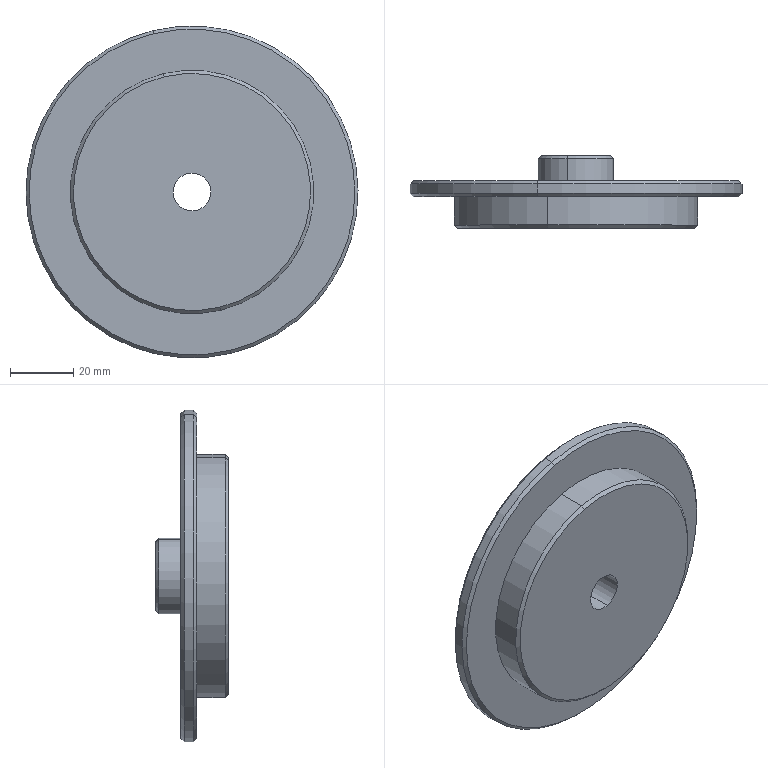Component | SolidWorks | RubberStopWheel-1 | 1 solid | 20 faces | box 105 x 23 x 105 mm | volume 90395 mm3 | cone 8 | cylinder 8 | plane 4 | commonest cylinder face diameters 12 x2 77 x2 105 x2 24 x2
build123d program:
from build123d import *

# Parameters (mm, degrees)
SKETCH1_R           = 12
BOSS_EXTRUDE1_DEPTH = 8
SKETCH2_R           = 52.5
BOSS_EXTRUDE2_DEPTH = 5
SKETCH3_R           = 38.5
BOSS_EXTRUDE3_DEPTH = 10
SKETCH4_R           = 6
CUT_EXTRUDE1_DEPTH  = 99
CHAMFER1_SIZE       = 1


with BuildPart() as part:
    # Sketch1 → Boss-Extrude1 (new body)
    with BuildSketch(Plane.XY):
        Circle(SKETCH1_R)
    extrude(amount=BOSS_EXTRUDE1_DEPTH)

    # Sketch2 → Boss-Extrude2 (add)
    with BuildSketch(Plane.XY.offset(8)):
        Circle(SKETCH2_R)
    extrude(amount=BOSS_EXTRUDE2_DEPTH)

    # Sketch3 → Boss-Extrude3 (add)
    with BuildSketch(Plane.XY.offset(13)):
        Circle(SKETCH3_R)
    extrude(amount=BOSS_EXTRUDE3_DEPTH)

    # Sketch4 → Cut-Extrude1 (cut)
    with BuildSketch(Plane.XY.offset(23)):
        Circle(SKETCH4_R)
    extrude(amount=-CUT_EXTRUDE1_DEPTH, mode=Mode.SUBTRACT)

    # Chamfer1
    chamfer1_edges = [part.edges().sort_by_distance(p)[0] for p in [
        (-38.5, 0, 23),
        (-12, 0, 0),
        (-52.5, 0, 8),
        (-52.5, 0, 13),
    ]]
    chamfer(chamfer1_edges, length=CHAMFER1_SIZE)


solid = part.part

# Placed as in the assembly
solid = solid.moved(Location((-48.547, -49.498, 328), (90, 0, 0)))
STEP:
#1=COLOUR_RGB('',0.7922,0.8196,0.9333);
#2=FILL_AREA_STYLE_COLOUR('',#1);
#3=FILL_AREA_STYLE('',(#2));
#4=SURFACE_STYLE_FILL_AREA(#3);
#5=SURFACE_SIDE_STYLE('',(#4));
#6=SURFACE_STYLE_USAGE(.BOTH.,#5);
#7=PRESENTATION_STYLE_ASSIGNMENT((#6));
#8=CARTESIAN_POINT('',(-1.565,-2.854,11.478));
#9=VERTEX_POINT('',#8);
#10=CARTESIAN_POINT('',(-2.257,-2.854,14.349));
#11=VERTEX_POINT('',#10);
#12=CARTESIAN_POINT('',(-1.911,-2.854,12.913));
#13=DIRECTION('',(0.,-1.,0.));
#14=DIRECTION('',(0.2342,0.,-0.9722));
#15=AXIS2_PLACEMENT_3D('',#12,#13,#14);
#16=CIRCLE('',#15,1.476);
#17=EDGE_CURVE('',#9,#11,#16,.T.);
#18=ORIENTED_EDGE('',*,*,#17,.F.);
#19=CARTESIAN_POINT('',(-1.556,-2.815,11.44));
#20=VERTEX_POINT('',#19);
#21=CARTESIAN_POINT('',(-1.565,-2.854,11.478));
#22=DIRECTION('',(0.1656,0.7071,-0.6874));
#23=VECTOR('',#22,39.37);
#24=LINE('',#21,#23);
#25=EDGE_CURVE('',#9,#20,#24,.T.);
#26=ORIENTED_EDGE('',*,*,#25,.T.);
#27=CARTESIAN_POINT('',(-2.266,-2.815,14.387));
#28=VERTEX_POINT('',#27);
#29=CARTESIAN_POINT('',(-1.911,-2.815,12.913));
#30=DIRECTION('',(-0.,1.,-0.));
#31=DIRECTION('',(0.2342,0.,-0.9722));
#32=AXIS2_PLACEMENT_3D('',#29,#30,#31);
#33=CIRCLE('',#32,1.516);
#34=EDGE_CURVE('',#28,#20,#33,.T.);
#35=ORIENTED_EDGE('',*,*,#34,.F.);
#36=CARTESIAN_POINT('',(-2.257,-2.854,14.349));
#37=DIRECTION('',(-0.1656,0.7071,0.6874));
#38=VECTOR('',#37,39.37);
#39=LINE('',#36,#38);
#40=EDGE_CURVE('',#11,#28,#39,.T.);
#41=ORIENTED_EDGE('',*,*,#40,.F.);
#42=EDGE_LOOP('',(#18,#26,#35,#41));
#43=FACE_OUTER_BOUND('',#42,.T.);
#44=CARTESIAN_POINT('',(-1.911,-2.854,12.913));
#45=DIRECTION('',(-0.,1.,-0.));
#46=DIRECTION('',(-0.2342,0.,0.9722));
#47=AXIS2_PLACEMENT_3D('',#44,#45,#46);
#48=CONICAL_SURFACE('',#47,1.476,0.7854);
#49=ADVANCED_FACE('',(#43),#48,.T.);
#50=CARTESIAN_POINT('',(-2.013,-1.949,13.334));
#51=VERTEX_POINT('',#50);
#52=CARTESIAN_POINT('',(-1.81,-1.949,12.492));
#53=VERTEX_POINT('',#52);
#54=CARTESIAN_POINT('',(-1.911,-1.949,12.913));
#55=DIRECTION('',(-0.,1.,-0.));
#56=DIRECTION('',(0.2342,0.,-0.9722));
#57=AXIS2_PLACEMENT_3D('',#54,#55,#56);
#58=CIRCLE('',#57,0.4331);
#59=EDGE_CURVE('',#51,#53,#58,.T.);
#60=ORIENTED_EDGE('',*,*,#59,.F.);
#61=CARTESIAN_POINT('',(-2.022,-1.988,13.373));
#62=VERTEX_POINT('',#61);
#63=CARTESIAN_POINT('',(-2.022,-1.988,13.373));
#64=DIRECTION('',(-0.1656,-0.7071,0.6874));
#65=VECTOR('',#64,39.37);
#66=LINE('',#63,#65);
#67=EDGE_CURVE('',#51,#62,#66,.T.);
#68=ORIENTED_EDGE('',*,*,#67,.T.);
#69=CARTESIAN_POINT('',(-1.801,-1.988,12.454));
#70=VERTEX_POINT('',#69);
#71=CARTESIAN_POINT('',(-1.911,-1.988,12.913));
#72=DIRECTION('',(0.,-1.,0.));
#73=DIRECTION('',(0.2342,0.,-0.9722));
#74=AXIS2_PLACEMENT_3D('',#71,#72,#73);
#75=CIRCLE('',#74,0.4724);
#76=EDGE_CURVE('',#70,#62,#75,.T.);
#77=ORIENTED_EDGE('',*,*,#76,.F.);
#78=CARTESIAN_POINT('',(-1.801,-1.988,12.454));
#79=DIRECTION('',(0.1656,-0.7071,-0.6874));
#80=VECTOR('',#79,39.37);
#81=LINE('',#78,#80);
#82=EDGE_CURVE('',#53,#70,#81,.T.);
#83=ORIENTED_EDGE('',*,*,#82,.F.);
#84=EDGE_LOOP('',(#60,#68,#77,#83));
#85=FACE_OUTER_BOUND('',#84,.T.);
#86=CARTESIAN_POINT('',(-1.911,-1.988,12.913));
#87=DIRECTION('',(0.,-1.,0.));
#88=DIRECTION('',(0.2342,0.,-0.9722));
#89=AXIS2_PLACEMENT_3D('',#86,#87,#88);
#90=CONICAL_SURFACE('',#89,0.4724,0.7854);
#91=ADVANCED_FACE('',(#85),#90,.T.);
#92=CARTESIAN_POINT('',(-1.436,-2.461,10.942));
#93=VERTEX_POINT('',#92);
#94=CARTESIAN_POINT('',(-2.386,-2.461,14.885));
#95=VERTEX_POINT('',#94);
#96=CARTESIAN_POINT('',(-1.911,-2.461,12.913));
#97=DIRECTION('',(0.,-1.,0.));
#98=DIRECTION('',(0.2342,0.,-0.9722));
#99=AXIS2_PLACEMENT_3D('',#96,#97,#98);
#100=CIRCLE('',#99,2.028);
#101=EDGE_CURVE('',#93,#95,#100,.T.);
#102=ORIENTED_EDGE('',*,*,#101,.F.);
#103=CARTESIAN_POINT('',(-1.427,-2.421,10.904));
#104=VERTEX_POINT('',#103);
#105=CARTESIAN_POINT('',(-1.436,-2.461,10.942));
#106=DIRECTION('',(0.1656,0.7071,-0.6874));
#107=VECTOR('',#106,39.37);
#108=LINE('',#105,#107);
#109=EDGE_CURVE('',#93,#104,#108,.T.);
#110=ORIENTED_EDGE('',*,*,#109,.T.);
#111=CARTESIAN_POINT('',(-2.395,-2.421,14.923));
#112=VERTEX_POINT('',#111);
#113=CARTESIAN_POINT('',(-1.911,-2.421,12.913));
#114=DIRECTION('',(-0.,1.,-0.));
#115=DIRECTION('',(0.2342,0.,-0.9722));
#116=AXIS2_PLACEMENT_3D('',#113,#114,#115);
#117=CIRCLE('',#116,2.067);
#118=EDGE_CURVE('',#112,#104,#117,.T.);
#119=ORIENTED_EDGE('',*,*,#118,.F.);
#120=CARTESIAN_POINT('',(-2.386,-2.461,14.885));
#121=DIRECTION('',(-0.1656,0.7071,0.6874));
#122=VECTOR('',#121,39.37);
#123=LINE('',#120,#122);
#124=EDGE_CURVE('',#95,#112,#123,.T.);
#125=ORIENTED_EDGE('',*,*,#124,.F.);
#126=EDGE_LOOP('',(#102,#110,#119,#125));
#127=FACE_OUTER_BOUND('',#126,.T.);
#128=CARTESIAN_POINT('',(-1.911,-2.461,12.913));
#129=DIRECTION('',(-0.,1.,-0.));
#130=DIRECTION('',(-0.2342,-0.,0.9722));
#131=AXIS2_PLACEMENT_3D('',#128,#129,#130);
#132=CONICAL_SURFACE('',#131,2.028,0.7854);
#133=ADVANCED_FACE('',(#127),#132,.T.);
#134=CARTESIAN_POINT('',(-2.386,-2.264,14.885));
#135=VERTEX_POINT('',#134);
#136=CARTESIAN_POINT('',(-1.436,-2.264,10.942));
#137=VERTEX_POINT('',#136);
#138=CARTESIAN_POINT('',(-1.911,-2.264,12.913));
#139=DIRECTION('',(-0.,1.,-0.));
#140=DIRECTION('',(0.2342,0.,-0.9722));
#141=AXIS2_PLACEMENT_3D('',#138,#139,#140);
#142=CIRCLE('',#141,2.028);
#143=EDGE_CURVE('',#135,#137,#142,.T.);
#144=ORIENTED_EDGE('',*,*,#143,.F.);
#145=CARTESIAN_POINT('',(-2.395,-2.303,14.923));
#146=VERTEX_POINT('',#145);
#147=CARTESIAN_POINT('',(-2.395,-2.303,14.923));
#148=DIRECTION('',(-0.1656,-0.7071,0.6874));
#149=VECTOR('',#148,39.37);
#150=LINE('',#147,#149);
#151=EDGE_CURVE('',#135,#146,#150,.T.);
#152=ORIENTED_EDGE('',*,*,#151,.T.);
#153=CARTESIAN_POINT('',(-1.427,-2.303,10.904));
#154=VERTEX_POINT('',#153);
#155=CARTESIAN_POINT('',(-1.911,-2.303,12.913));
#156=DIRECTION('',(0.,-1.,0.));
#157=DIRECTION('',(0.2342,0.,-0.9722));
#158=AXIS2_PLACEMENT_3D('',#155,#156,#157);
#159=CIRCLE('',#158,2.067);
#160=EDGE_CURVE('',#154,#146,#159,.T.);
#161=ORIENTED_EDGE('',*,*,#160,.F.);
#162=CARTESIAN_POINT('',(-1.427,-2.303,10.904));
#163=DIRECTION('',(0.1656,-0.7071,-0.6874));
#164=VECTOR('',#163,39.37);
#165=LINE('',#162,#164);
#166=EDGE_CURVE('',#137,#154,#165,.T.);
#167=ORIENTED_EDGE('',*,*,#166,.F.);
#168=EDGE_LOOP('',(#144,#152,#161,#167));
#169=FACE_OUTER_BOUND('',#168,.T.);
#170=CARTESIAN_POINT('',(-1.911,-2.303,12.913));
#171=DIRECTION('',(0.,-1.,0.));
#172=DIRECTION('',(0.2342,0.,-0.9722));
#173=AXIS2_PLACEMENT_3D('',#170,#171,#172);
#174=CONICAL_SURFACE('',#173,2.067,0.7854);
#175=ADVANCED_FACE('',(#169),#174,.T.);
#176=CARTESIAN_POINT('',(-1.967,-1.949,13.143));
#177=VERTEX_POINT('',#176);
#178=CARTESIAN_POINT('',(-1.856,-1.949,12.684));
#179=VERTEX_POINT('',#178);
#180=CARTESIAN_POINT('',(-1.911,-1.949,12.913));
#181=DIRECTION('',(0.,-1.,0.));
#182=DIRECTION('',(0.2342,0.,-0.9722));
#183=AXIS2_PLACEMENT_3D('',#180,#181,#182);
#184=CIRCLE('',#183,0.2362);
#185=EDGE_CURVE('',#177,#179,#184,.T.);
#186=ORIENTED_EDGE('',*,*,#185,.F.);
#187=CARTESIAN_POINT('',(-1.967,-2.854,13.143));
#188=VERTEX_POINT('',#187);
#189=CARTESIAN_POINT('',(-1.967,1.043,13.143));
#190=DIRECTION('',(0.,-1.,0.));
#191=VECTOR('',#190,39.37);
#192=LINE('',#189,#191);
#193=EDGE_CURVE('',#177,#188,#192,.T.);
#194=ORIENTED_EDGE('',*,*,#193,.T.);
#195=CARTESIAN_POINT('',(-1.856,-2.854,12.684));
#196=VERTEX_POINT('',#195);
#197=CARTESIAN_POINT('',(-1.911,-2.854,12.913));
#198=DIRECTION('',(0.,-1.,0.));
#199=DIRECTION('',(0.2342,0.,-0.9722));
#200=AXIS2_PLACEMENT_3D('',#197,#198,#199);
#201=CIRCLE('',#200,0.2362);
#202=EDGE_CURVE('',#188,#196,#201,.T.);
#203=ORIENTED_EDGE('',*,*,#202,.T.);
#204=CARTESIAN_POINT('',(-1.856,1.043,12.684));
#205=DIRECTION('',(0.,-1.,0.));
#206=VECTOR('',#205,39.37);
#207=LINE('',#204,#206);
#208=EDGE_CURVE('',#179,#196,#207,.T.);
#209=ORIENTED_EDGE('',*,*,#208,.F.);
#210=EDGE_LOOP('',(#186,#194,#203,#209));
#211=FACE_OUTER_BOUND('',#210,.T.);
#212=CARTESIAN_POINT('',(-1.911,1.043,12.913));
#213=DIRECTION('',(0.,-1.,0.));
#214=DIRECTION('',(0.2342,0.,-0.9722));
#215=AXIS2_PLACEMENT_3D('',#212,#213,#214);
#216=CYLINDRICAL_SURFACE('',#215,0.2362);
#217=ADVANCED_FACE('',(#211),#216,.F.);
#218=ORIENTED_EDGE('',*,*,#34,.T.);
#219=CARTESIAN_POINT('',(-1.556,-2.461,11.44));
#220=VERTEX_POINT('',#219);
#221=CARTESIAN_POINT('',(-1.556,-2.854,11.44));
#222=DIRECTION('',(-0.,1.,-0.));
#223=VECTOR('',#222,39.37);
#224=LINE('',#221,#223);
#225=EDGE_CURVE('',#20,#220,#224,.T.);
#226=ORIENTED_EDGE('',*,*,#225,.T.);
#227=CARTESIAN_POINT('',(-2.266,-2.461,14.387));
#228=VERTEX_POINT('',#227);
#229=CARTESIAN_POINT('',(-1.911,-2.461,12.913));
#230=DIRECTION('',(0.,-1.,0.));
#231=DIRECTION('',(0.2342,0.,-0.9722));
#232=AXIS2_PLACEMENT_3D('',#229,#230,#231);
#233=CIRCLE('',#232,1.516);
#234=EDGE_CURVE('',#220,#228,#233,.T.);
#235=ORIENTED_EDGE('',*,*,#234,.T.);
#236=CARTESIAN_POINT('',(-2.266,-2.854,14.387));
#237=DIRECTION('',(-0.,1.,-0.));
#238=VECTOR('',#237,39.37);
#239=LINE('',#236,#238);
#240=EDGE_CURVE('',#28,#228,#239,.T.);
#241=ORIENTED_EDGE('',*,*,#240,.F.);
#242=EDGE_LOOP('',(#218,#226,#235,#241));
#243=FACE_OUTER_BOUND('',#242,.T.);
#244=CARTESIAN_POINT('',(-1.911,-2.854,12.913));
#245=DIRECTION('',(-0.,1.,-0.));
#246=DIRECTION('',(-0.2342,0.,0.9722));
#247=AXIS2_PLACEMENT_3D('',#244,#245,#246);
#248=CYLINDRICAL_SURFACE('',#247,1.516);
#249=ADVANCED_FACE('',(#243),#248,.T.);
#250=ORIENTED_EDGE('',*,*,#118,.T.);
#251=CARTESIAN_POINT('',(-1.427,-2.461,10.904));
#252=DIRECTION('',(-0.,1.,-0.));
#253=VECTOR('',#252,39.37);
#254=LINE('',#251,#253);
#255=EDGE_CURVE('',#104,#154,#254,.T.);
#256=ORIENTED_EDGE('',*,*,#255,.T.);
#257=ORIENTED_EDGE('',*,*,#160,.T.);
#258=CARTESIAN_POINT('',(-2.395,-2.461,14.923));
#259=DIRECTION('',(-0.,1.,-0.));
#260=VECTOR('',#259,39.37);
#261=LINE('',#258,#260);
#262=EDGE_CURVE('',#112,#146,#261,.T.);
#263=ORIENTED_EDGE('',*,*,#262,.F.);
#264=EDGE_LOOP('',(#250,#256,#257,#263));
#265=FACE_OUTER_BOUND('',#264,.T.);
#266=CARTESIAN_POINT('',(-1.911,-2.461,12.913));
#267=DIRECTION('',(-0.,1.,-0.));
#268=DIRECTION('',(-0.2342,-0.,0.9722));
#269=AXIS2_PLACEMENT_3D('',#266,#267,#268);
#270=CYLINDRICAL_SURFACE('',#269,2.067);
#271=ADVANCED_FACE('',(#265),#270,.T.);
#272=CARTESIAN_POINT('',(-1.801,-2.264,12.454));
#273=VERTEX_POINT('',#272);
#274=CARTESIAN_POINT('',(-2.022,-2.264,13.373));
#275=VERTEX_POINT('',#274);
#276=CARTESIAN_POINT('',(-1.911,-2.264,12.913));
#277=DIRECTION('',(0.,-1.,0.));
#278=DIRECTION('',(0.2342,0.,-0.9722));
#279=AXIS2_PLACEMENT_3D('',#276,#277,#278);
#280=CIRCLE('',#279,0.4724);
#281=EDGE_CURVE('',#273,#275,#280,.T.);
#282=ORIENTED_EDGE('',*,*,#281,.F.);
#283=CARTESIAN_POINT('',(-1.801,-2.264,12.454));
#284=DIRECTION('',(-0.,1.,-0.));
#285=VECTOR('',#284,39.37);
#286=LINE('',#283,#285);
#287=EDGE_CURVE('',#273,#70,#286,.T.);
#288=ORIENTED_EDGE('',*,*,#287,.T.);
#289=ORIENTED_EDGE('',*,*,#76,.T.);
#290=CARTESIAN_POINT('',(-2.022,-2.264,13.373));
#291=DIRECTION('',(-0.,1.,-0.));
#292=VECTOR('',#291,39.37);
#293=LINE('',#290,#292);
#294=EDGE_CURVE('',#275,#62,#293,.T.);
#295=ORIENTED_EDGE('',*,*,#294,.F.);
#296=EDGE_LOOP('',(#282,#288,#289,#295));
#297=FACE_OUTER_BOUND('',#296,.T.);
#298=CARTESIAN_POINT('',(-1.911,-2.264,12.913));
#299=DIRECTION('',(-0.,1.,-0.));
#300=DIRECTION('',(-0.2342,0.,0.9722));
#301=AXIS2_PLACEMENT_3D('',#298,#299,#300);
#302=CYLINDRICAL_SURFACE('',#301,0.4724);
#303=ADVANCED_FACE('',(#297),#302,.T.);
#304=ORIENTED_EDGE('',*,*,#287,.F.);
#305=CARTESIAN_POINT('',(-1.911,-2.264,12.913));
#306=DIRECTION('',(0.,-1.,0.));
#307=DIRECTION('',(0.2342,0.,-0.9722));
#308=AXIS2_PLACEMENT_3D('',#305,#306,#307);
#309=CIRCLE('',#308,0.4724);
#310=EDGE_CURVE('',#275,#273,#309,.T.);
#311=ORIENTED_EDGE('',*,*,#310,.F.);
#312=ORIENTED_EDGE('',*,*,#294,.T.);
#313=CARTESIAN_POINT('',(-1.911,-1.988,12.913));
#314=DIRECTION('',(0.,-1.,0.));
#315=DIRECTION('',(0.2342,0.,-0.9722));
#316=AXIS2_PLACEMENT_3D('',#313,#314,#315);
#317=CIRCLE('',#316,0.4724);
#318=EDGE_CURVE('',#62,#70,#317,.T.);
#319=ORIENTED_EDGE('',*,*,#318,.T.);
#320=EDGE_LOOP('',(#304,#311,#312,#319));
#321=FACE_OUTER_BOUND('',#320,.T.);
#322=CARTESIAN_POINT('',(-1.911,-2.264,12.913));
#323=DIRECTION('',(-0.,1.,-0.));
#324=DIRECTION('',(-0.2342,0.,0.9722));
#325=AXIS2_PLACEMENT_3D('',#322,#323,#324);
#326=CYLINDRICAL_SURFACE('',#325,0.4724);
#327=ADVANCED_FACE('',(#321),#326,.T.);
#328=CARTESIAN_POINT('',(-1.911,-1.949,12.913));
#329=DIRECTION('',(-0.,1.,-0.));
#330=DIRECTION('',(0.2342,0.,-0.9722));
#331=AXIS2_PLACEMENT_3D('',#328,#329,#330);
#332=CIRCLE('',#331,0.4331);
#333=EDGE_CURVE('',#53,#51,#332,.T.);
#334=ORIENTED_EDGE('',*,*,#333,.T.);
#335=ORIENTED_EDGE('',*,*,#59,.T.);
#336=EDGE_LOOP('',(#334,#335));
#337=FACE_OUTER_BOUND('',#336,.T.);
#338=CARTESIAN_POINT('',(-1.911,-1.949,12.913));
#339=DIRECTION('',(0.,-1.,0.));
#340=DIRECTION('',(0.2342,0.,-0.9722));
#341=AXIS2_PLACEMENT_3D('',#338,#339,#340);
#342=CIRCLE('',#341,0.2362);
#343=EDGE_CURVE('',#179,#177,#342,.T.);
#344=ORIENTED_EDGE('',*,*,#343,.T.);
#345=ORIENTED_EDGE('',*,*,#185,.T.);
#346=EDGE_LOOP('',(#344,#345));
#347=FACE_BOUND('',#346,.T.);
#348=CARTESIAN_POINT('',(-1.911,-1.949,12.913));
#349=DIRECTION('',(0.,-1.,0.));
#350=DIRECTION('',(0.2342,0.,-0.9722));
#351=AXIS2_PLACEMENT_3D('',#348,#349,#350);
#352=PLANE('',#351);
#353=ADVANCED_FACE('',(#337,#347),#352,.F.);
#354=ORIENTED_EDGE('',*,*,#255,.F.);
#355=CARTESIAN_POINT('',(-1.911,-2.421,12.913));
#356=DIRECTION('',(-0.,1.,-0.));
#357=DIRECTION('',(0.2342,0.,-0.9722));
#358=AXIS2_PLACEMENT_3D('',#355,#356,#357);
#359=CIRCLE('',#358,2.067);
#360=EDGE_CURVE('',#104,#112,#359,.T.);
#361=ORIENTED_EDGE('',*,*,#360,.T.);
#362=ORIENTED_EDGE('',*,*,#262,.T.);
#363=CARTESIAN_POINT('',(-1.911,-2.303,12.913));
#364=DIRECTION('',(0.,-1.,0.));
#365=DIRECTION('',(0.2342,0.,-0.9722));
#366=AXIS2_PLACEMENT_3D('',#363,#364,#365);
#367=CIRCLE('',#366,2.067);
#368=EDGE_CURVE('',#146,#154,#367,.T.);
#369=ORIENTED_EDGE('',*,*,#368,.T.);
#370=EDGE_LOOP('',(#354,#361,#362,#369));
#371=FACE_OUTER_BOUND('',#370,.T.);
#372=CARTESIAN_POINT('',(-1.911,-2.461,12.913));
#373=DIRECTION('',(-0.,1.,-0.));
#374=DIRECTION('',(-0.2342,-0.,0.9722));
#375=AXIS2_PLACEMENT_3D('',#372,#373,#374);
#376=CYLINDRICAL_SURFACE('',#375,2.067);
#377=ADVANCED_FACE('',(#371),#376,.T.);
#378=CARTESIAN_POINT('',(-1.911,-2.461,12.913));
#379=DIRECTION('',(0.,-1.,0.));
#380=DIRECTION('',(0.2342,0.,-0.9722));
#381=AXIS2_PLACEMENT_3D('',#378,#379,#380);
#382=CIRCLE('',#381,2.028);
#383=EDGE_CURVE('',#95,#93,#382,.T.);
#384=ORIENTED_EDGE('',*,*,#383,.T.);
#385=ORIENTED_EDGE('',*,*,#101,.T.);
#386=EDGE_LOOP('',(#384,#385));
#387=FACE_OUTER_BOUND('',#386,.T.);
#388=CARTESIAN_POINT('',(-1.911,-2.461,12.913));
#389=DIRECTION('',(0.,-1.,0.));
#390=DIRECTION('',(0.2342,0.,-0.9722));
#391=AXIS2_PLACEMENT_3D('',#388,#389,#390);
#392=CIRCLE('',#391,1.516);
#393=EDGE_CURVE('',#228,#220,#392,.T.);
#394=ORIENTED_EDGE('',*,*,#393,.F.);
#395=ORIENTED_EDGE('',*,*,#234,.F.);
#396=EDGE_LOOP('',(#394,#395));
#397=FACE_BOUND('',#396,.T.);
#398=CARTESIAN_POINT('',(-1.911,-2.461,12.913));
#399=DIRECTION('',(0.,-1.,0.));
#400=DIRECTION('',(0.2342,0.,-0.9722));
#401=AXIS2_PLACEMENT_3D('',#398,#399,#400);
#402=PLANE('',#401);
#403=ADVANCED_FACE('',(#387,#397),#402,.T.);
#404=CARTESIAN_POINT('',(-1.911,-2.264,12.913));
#405=DIRECTION('',(-0.,1.,-0.));
#406=DIRECTION('',(0.2342,0.,-0.9722));
#407=AXIS2_PLACEMENT_3D('',#404,#405,#406);
#408=CIRCLE('',#407,2.028);
#409=EDGE_CURVE('',#137,#135,#408,.T.);
#410=ORIENTED_EDGE('',*,*,#409,.T.);
#411=ORIENTED_EDGE('',*,*,#143,.T.);
#412=EDGE_LOOP('',(#410,#411));
#413=FACE_OUTER_BOUND('',#412,.T.);
#414=ORIENTED_EDGE('',*,*,#310,.T.);
#415=ORIENTED_EDGE('',*,*,#281,.T.);
#416=EDGE_LOOP('',(#414,#415));
#417=FACE_BOUND('',#416,.T.);
#418=CARTESIAN_POINT('',(-1.911,-2.264,12.913));
#419=DIRECTION('',(0.,-1.,0.));
#420=DIRECTION('',(0.2342,0.,-0.9722));
#421=AXIS2_PLACEMENT_3D('',#418,#419,#420);
#422=PLANE('',#421);
#423=ADVANCED_FACE('',(#413,#417),#422,.F.);
#424=ORIENTED_EDGE('',*,*,#225,.F.);
#425=CARTESIAN_POINT('',(-1.911,-2.815,12.913));
#426=DIRECTION('',(-0.,1.,-0.));
#427=DIRECTION('',(0.2342,0.,-0.9722));
#428=AXIS2_PLACEMENT_3D('',#425,#426,#427);
#429=CIRCLE('',#428,1.516);
#430=EDGE_CURVE('',#20,#28,#429,.T.);
#431=ORIENTED_EDGE('',*,*,#430,.T.);
#432=ORIENTED_EDGE('',*,*,#240,.T.);
#433=ORIENTED_EDGE('',*,*,#393,.T.);
#434=EDGE_LOOP('',(#424,#431,#432,#433));
#435=FACE_OUTER_BOUND('',#434,.T.);
#436=CARTESIAN_POINT('',(-1.911,-2.854,12.913));
#437=DIRECTION('',(-0.,1.,-0.));
#438=DIRECTION('',(-0.2342,0.,0.9722));
#439=AXIS2_PLACEMENT_3D('',#436,#437,#438);
#440=CYLINDRICAL_SURFACE('',#439,1.516);
#441=ADVANCED_FACE('',(#435),#440,.T.);
#442=CARTESIAN_POINT('',(-1.911,-2.854,12.913));
#443=DIRECTION('',(0.,-1.,0.));
#444=DIRECTION('',(0.2342,0.,-0.9722));
#445=AXIS2_PLACEMENT_3D('',#442,#443,#444);
#446=CIRCLE('',#445,1.476);
#447=EDGE_CURVE('',#11,#9,#446,.T.);
#448=ORIENTED_EDGE('',*,*,#447,.T.);
#449=ORIENTED_EDGE('',*,*,#17,.T.);
#450=EDGE_LOOP('',(#448,#449));
#451=FACE_OUTER_BOUND('',#450,.T.);
#452=CARTESIAN_POINT('',(-1.911,-2.854,12.913));
#453=DIRECTION('',(0.,-1.,0.));
#454=DIRECTION('',(0.2342,0.,-0.9722));
#455=AXIS2_PLACEMENT_3D('',#452,#453,#454);
#456=CIRCLE('',#455,0.2362);
#457=EDGE_CURVE('',#196,#188,#456,.T.);
#458=ORIENTED_EDGE('',*,*,#457,.F.);
#459=ORIENTED_EDGE('',*,*,#202,.F.);
#460=EDGE_LOOP('',(#458,#459));
#461=FACE_BOUND('',#460,.T.);
#462=CARTESIAN_POINT('',(-1.911,-2.854,12.913));
#463=DIRECTION('',(0.,-1.,0.));
#464=DIRECTION('',(0.2342,0.,-0.9722));
#465=AXIS2_PLACEMENT_3D('',#462,#463,#464);
#466=PLANE('',#465);
#467=ADVANCED_FACE('',(#451,#461),#466,.T.);
#468=ORIENTED_EDGE('',*,*,#193,.F.);
#469=ORIENTED_EDGE('',*,*,#343,.F.);
#470=ORIENTED_EDGE('',*,*,#208,.T.);
#471=ORIENTED_EDGE('',*,*,#457,.T.);
#472=EDGE_LOOP('',(#468,#469,#470,#471));
#473=FACE_OUTER_BOUND('',#472,.T.);
#474=CARTESIAN_POINT('',(-1.911,1.043,12.913));
#475=DIRECTION('',(0.,-1.,0.));
#476=DIRECTION('',(0.2342,0.,-0.9722));
#477=AXIS2_PLACEMENT_3D('',#474,#475,#476);
#478=CYLINDRICAL_SURFACE('',#477,0.2362);
#479=ADVANCED_FACE('',(#473),#478,.F.);
#480=ORIENTED_EDGE('',*,*,#151,.F.);
#481=ORIENTED_EDGE('',*,*,#409,.F.);
#482=ORIENTED_EDGE('',*,*,#166,.T.);
#483=ORIENTED_EDGE('',*,*,#368,.F.);
#484=EDGE_LOOP('',(#480,#481,#482,#483));
#485=FACE_OUTER_BOUND('',#484,.T.);
#486=CARTESIAN_POINT('',(-1.911,-2.303,12.913));
#487=DIRECTION('',(0.,-1.,0.));
#488=DIRECTION('',(0.2342,0.,-0.9722));
#489=AXIS2_PLACEMENT_3D('',#486,#487,#488);
#490=CONICAL_SURFACE('',#489,2.067,0.7854);
#491=ADVANCED_FACE('',(#485),#490,.T.);
#492=ORIENTED_EDGE('',*,*,#109,.F.);
#493=ORIENTED_EDGE('',*,*,#383,.F.);
#494=ORIENTED_EDGE('',*,*,#124,.T.);
#495=ORIENTED_EDGE('',*,*,#360,.F.);
#496=EDGE_LOOP('',(#492,#493,#494,#495));
#497=FACE_OUTER_BOUND('',#496,.T.);
#498=CARTESIAN_POINT('',(-1.911,-2.461,12.913));
#499=DIRECTION('',(-0.,1.,-0.));
#500=DIRECTION('',(-0.2342,-0.,0.9722));
#501=AXIS2_PLACEMENT_3D('',#498,#499,#500);
#502=CONICAL_SURFACE('',#501,2.028,0.7854);
#503=ADVANCED_FACE('',(#497),#502,.T.);
#504=ORIENTED_EDGE('',*,*,#67,.F.);
#505=ORIENTED_EDGE('',*,*,#333,.F.);
#506=ORIENTED_EDGE('',*,*,#82,.T.);
#507=ORIENTED_EDGE('',*,*,#318,.F.);
#508=EDGE_LOOP('',(#504,#505,#506,#507));
#509=FACE_OUTER_BOUND('',#508,.T.);
#510=CARTESIAN_POINT('',(-1.911,-1.988,12.913));
#511=DIRECTION('',(0.,-1.,0.));
#512=DIRECTION('',(0.2342,0.,-0.9722));
#513=AXIS2_PLACEMENT_3D('',#510,#511,#512);
#514=CONICAL_SURFACE('',#513,0.4724,0.7854);
#515=ADVANCED_FACE('',(#509),#514,.T.);
#516=ORIENTED_EDGE('',*,*,#25,.F.);
#517=ORIENTED_EDGE('',*,*,#447,.F.);
#518=ORIENTED_EDGE('',*,*,#40,.T.);
#519=ORIENTED_EDGE('',*,*,#430,.F.);
#520=EDGE_LOOP('',(#516,#517,#518,#519));
#521=FACE_OUTER_BOUND('',#520,.T.);
#522=CARTESIAN_POINT('',(-1.911,-2.854,12.913));
#523=DIRECTION('',(-0.,1.,-0.));
#524=DIRECTION('',(-0.2342,0.,0.9722));
#525=AXIS2_PLACEMENT_3D('',#522,#523,#524);
#526=CONICAL_SURFACE('',#525,1.476,0.7854);
#527=ADVANCED_FACE('',(#521),#526,.T.);
#528=CLOSED_SHELL('',(#49,#91,#133,#175,#217,#249,#271,#303,#327,#353,#377,#403,#423,#441,#467,#479,#491,#503,#515,#527));
#529=MANIFOLD_SOLID_BREP('',#528);
#530=STYLED_ITEM('',(#7),#529);
#531=(LENGTH_UNIT()NAMED_UNIT(*)SI_UNIT($,.METRE.));
#532=LENGTH_MEASURE_WITH_UNIT(LENGTH_MEASURE(0.0254),#531);
#533=DIMENSIONAL_EXPONENTS(1.,0.,0.,0.,0.,0.,0.);
#534=(CONVERSION_BASED_UNIT('',#532)LENGTH_UNIT()NAMED_UNIT(#533));
#535=UNCERTAINTY_MEASURE_WITH_UNIT(LENGTH_MEASURE(0.00001),#534,'','');
#536=(NAMED_UNIT(*)PLANE_ANGLE_UNIT()SI_UNIT($,.RADIAN.));
#537=(NAMED_UNIT(*)SI_UNIT($,.STERADIAN.)SOLID_ANGLE_UNIT());
#538=(GEOMETRIC_REPRESENTATION_CONTEXT(3)GLOBAL_UNCERTAINTY_ASSIGNED_CONTEXT((#535))GLOBAL_UNIT_ASSIGNED_CONTEXT((#534,#536,#537))REPRESENTATION_CONTEXT('',''));
#539=MECHANICAL_DESIGN_GEOMETRIC_PRESENTATION_REPRESENTATION('',(#530),#538);
#540=PRESENTATION_LAYER_ASSIGNMENT('','',(#530));
#541=CARTESIAN_POINT('',(0.,0.,0.));
#542=DIRECTION('',(0.,0.,1.));
#543=DIRECTION('',(1.,0.,0.));
#544=AXIS2_PLACEMENT_3D('',#541,#542,#543);
#545=(LENGTH_UNIT()NAMED_UNIT(*)SI_UNIT($,.METRE.));
#546=LENGTH_MEASURE_WITH_UNIT(LENGTH_MEASURE(0.0254),#545);
#547=DIMENSIONAL_EXPONENTS(1.,0.,0.,0.,0.,0.,0.);
#548=(CONVERSION_BASED_UNIT('',#546)LENGTH_UNIT()NAMED_UNIT(#547));
#549=UNCERTAINTY_MEASURE_WITH_UNIT(LENGTH_MEASURE(0.00001),#548,'','');
#550=(NAMED_UNIT(*)PLANE_ANGLE_UNIT()SI_UNIT($,.RADIAN.));
#551=(NAMED_UNIT(*)SI_UNIT($,.STERADIAN.)SOLID_ANGLE_UNIT());
#552=(GEOMETRIC_REPRESENTATION_CONTEXT(3)GLOBAL_UNCERTAINTY_ASSIGNED_CONTEXT((#549))GLOBAL_UNIT_ASSIGNED_CONTEXT((#548,#550,#551))REPRESENTATION_CONTEXT('',''));
#553=ADVANCED_BREP_SHAPE_REPRESENTATION('',(#529,#544),#552);